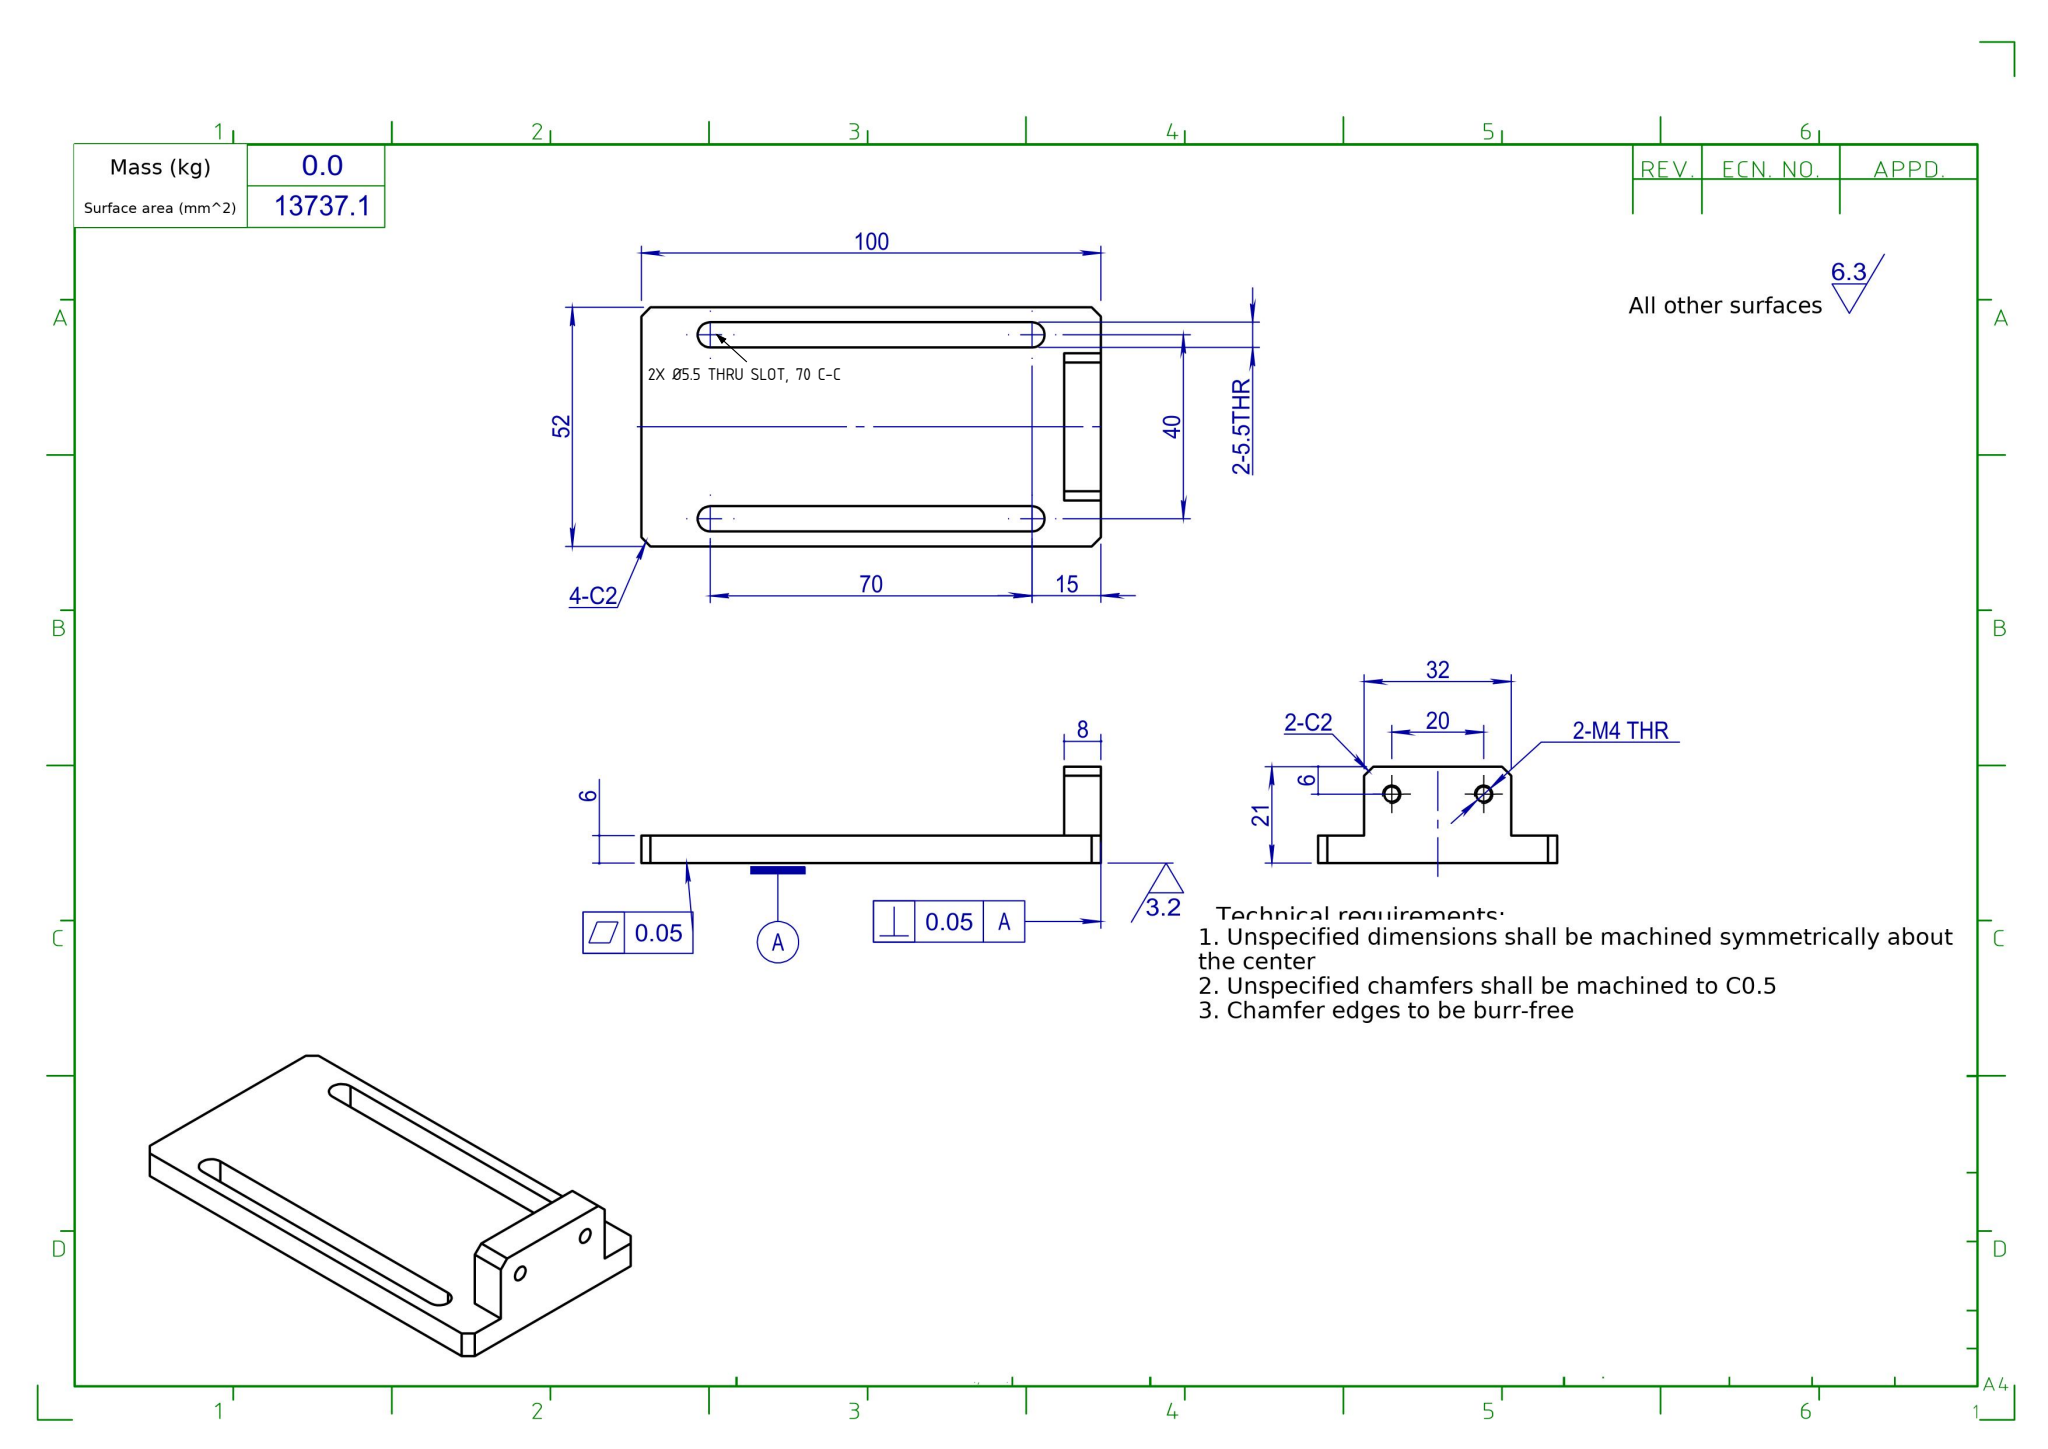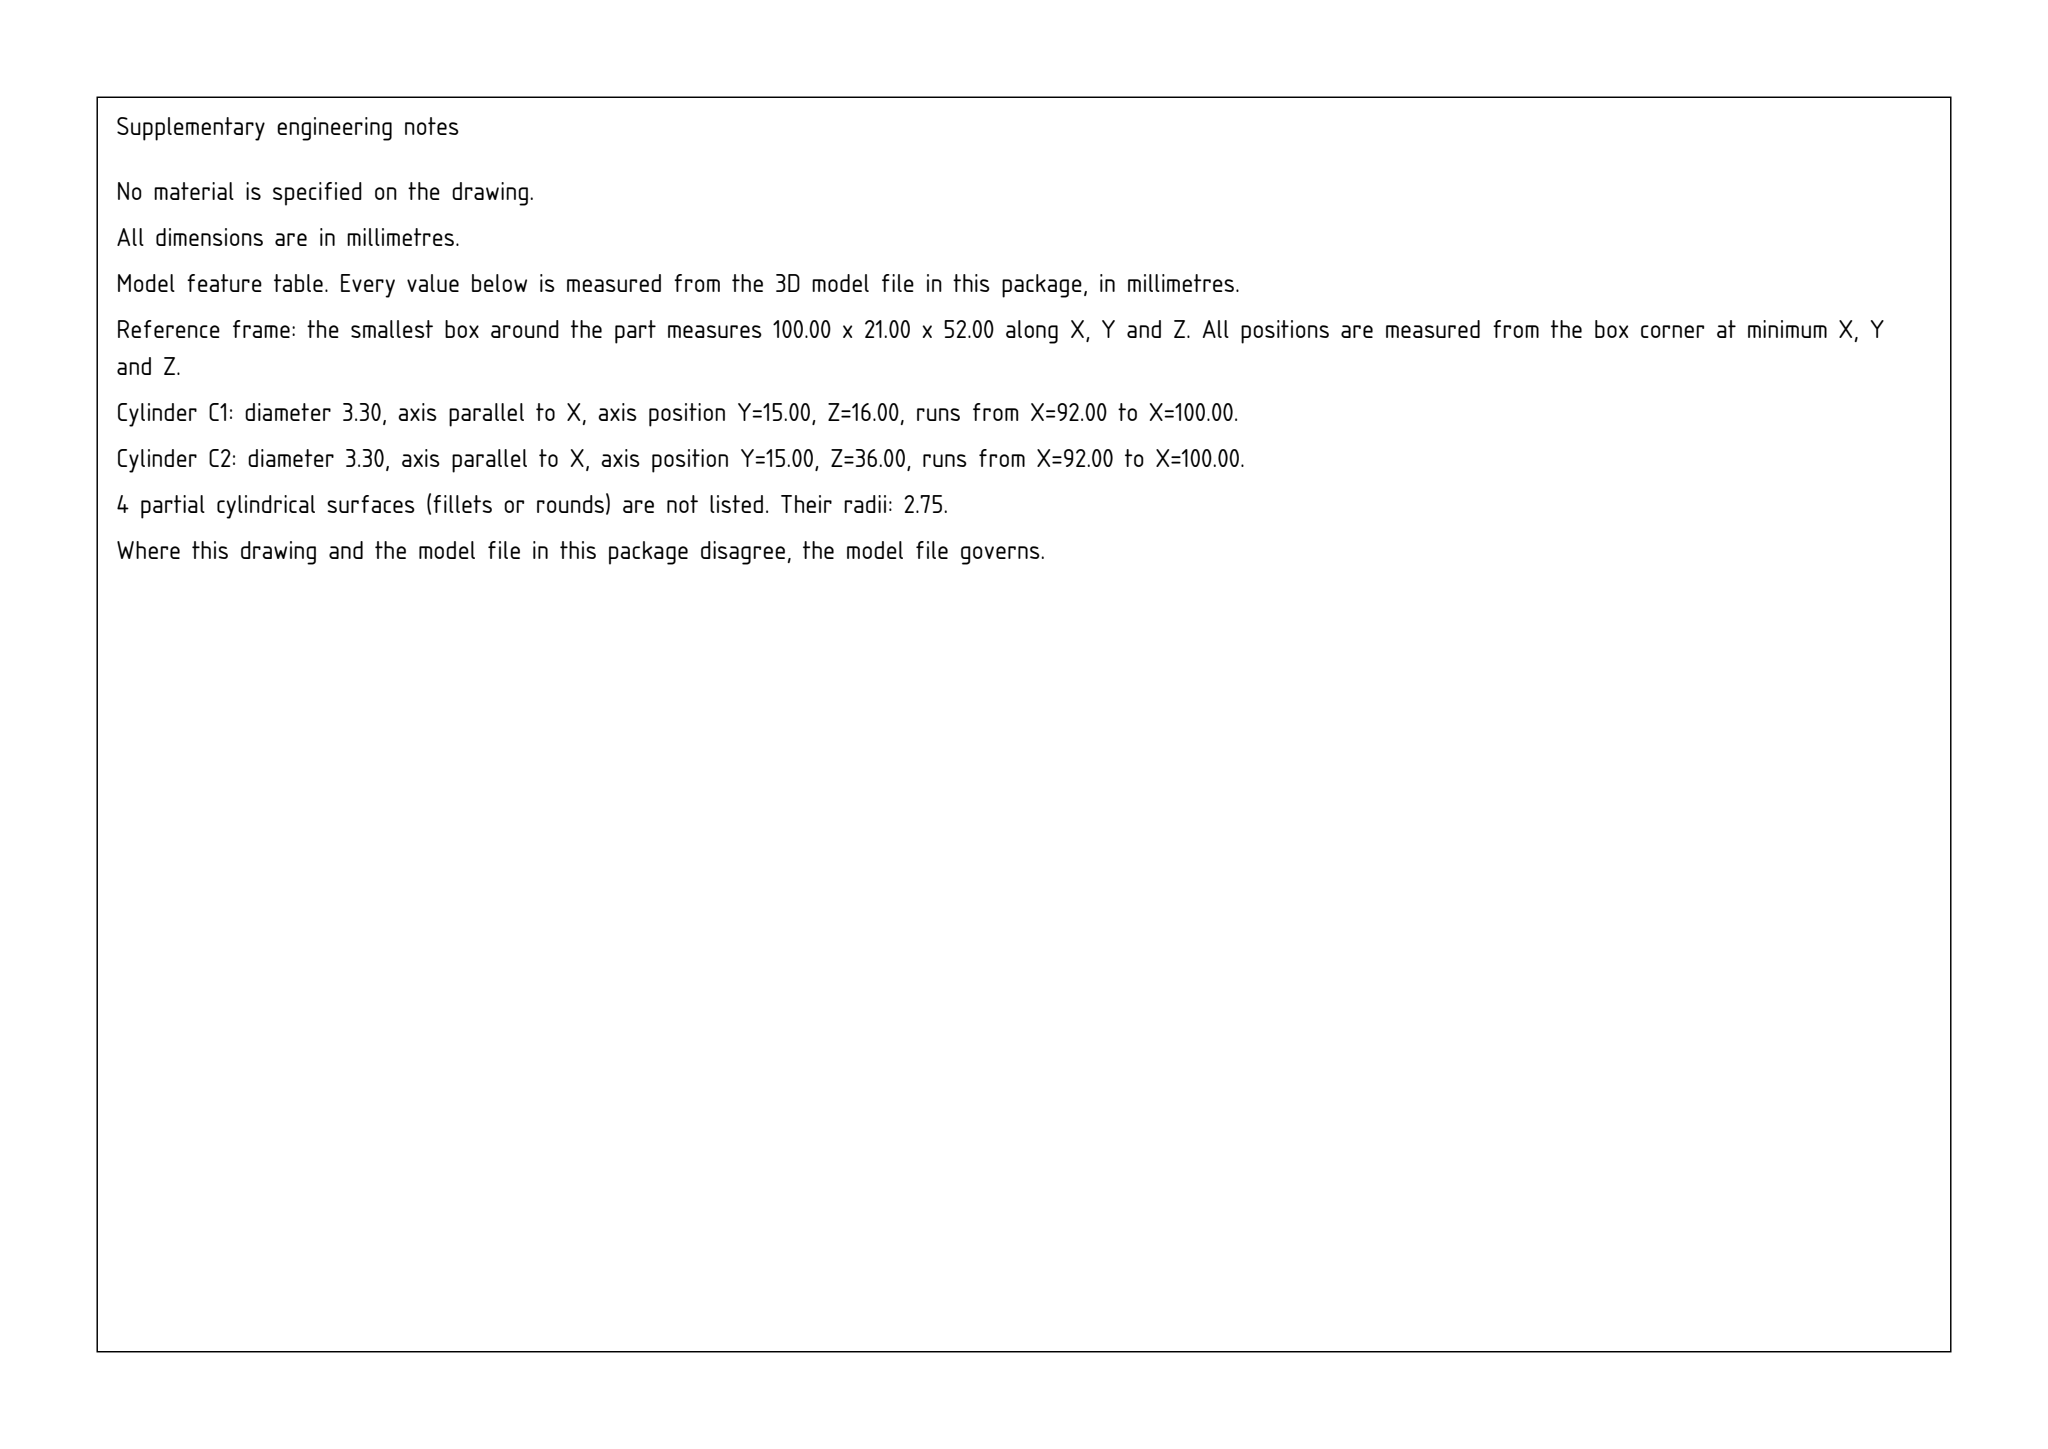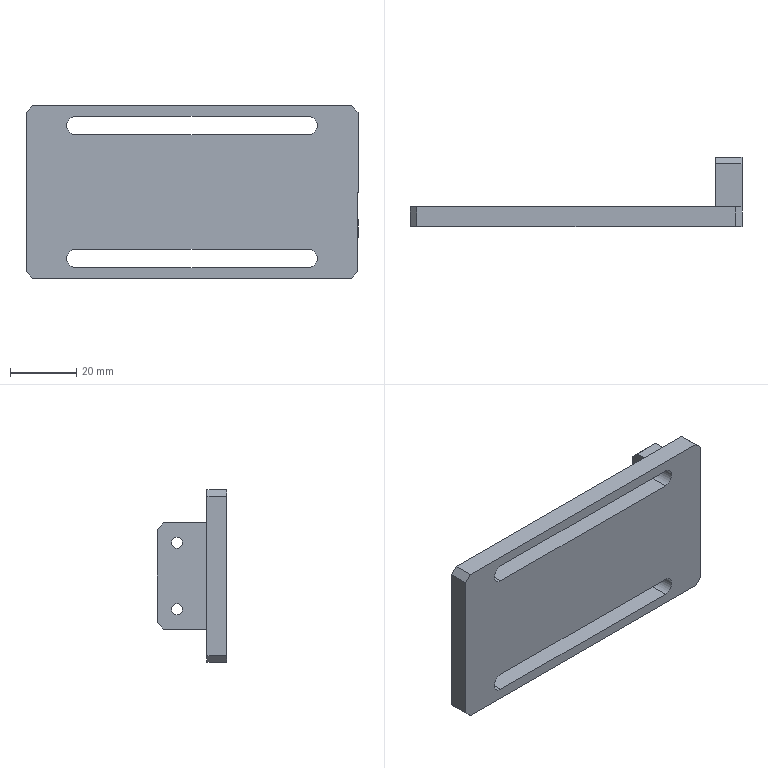Part | SolidWorks | mm | 1 solid | 28 faces | box 100 x 21 x 52 mm | volume 29918 mm3 | plane 20 | cylinder 8 | commonest cylinder face diameters 3.3 x4 5.5 x4
Drawing notes:
2-Ø5.5 THRU SLOTS, 70 LG C-C, SYM ABT CL | from the solid: Four 180° arcs Ø5.5 axis Y at x=15 & 85, z=6 & 46, from y=0 to 6 (thru 6 thk plate); slot ends 70 apart
build123d program:
from build123d import *

# Parameters (mm, degrees)
SKETCH1_W          = 100
SKETCH1_H          = 52
EXTRUDE1_DEPTH     = 3
SKETCH4_W          = 8
SKETCH4_H          = 52
EXTRUDE2_DEPTH     = 15
M4_TAPPED_HOLE1_D  = 3.3
CHAMFER1_SIZE      = 2
SKETCH9_W          = 10
SKETCH9_H          = 15
CUT_EXTRUDE3_DEPTH = 10
CHAMFER2_SIZE      = 2
CUT_EXTRUDE4_DEPTH = 59.318


with BuildPart() as part:
    # Sketch1 → Extrude1 (new, symmetric)
    with BuildSketch(Plane(origin=(0, 0, 0), x_dir=(1, 0, 0), z_dir=(0, 1, 0))):
        Rectangle(SKETCH1_W, SKETCH1_H)
    extrude(amount=EXTRUDE1_DEPTH, both=True)

    # Sketch4 → Extrude2 (add)
    with BuildSketch(Plane(origin=(0, 3, 0), x_dir=(1, 0, 0), z_dir=(0, 1, 0))):
        with Locations((46, 0)):
            Rectangle(SKETCH4_W, SKETCH4_H)
    extrude(amount=EXTRUDE2_DEPTH)

    # M4 Tapped Hole1 (through all)
    with Locations(Plane.ZY.offset(-42)):
        with Locations((-10, 12), (10, 12)):
            Hole(M4_TAPPED_HOLE1_D / 2)

    # Chamfer1
    chamfer1_edges = [part.edges().sort_by_distance(p)[0] for p in [
        (-50, 0, -26),
        (-50, 0, 26),
        (46, 18, 26),
        (46, 18, -26),
    ]]
    chamfer(chamfer1_edges, length=CHAMFER1_SIZE)

    # Sketch9 → Cut-Extrude3 (cut)
    with BuildSketch(Plane.ZY.offset(-42)):
        with Locations((-21, 10.5)):
            Rectangle(SKETCH9_W, SKETCH9_H)
        with Locations((21, 10.5)):
            Rectangle(SKETCH9_W, SKETCH9_H)
    extrude(amount=-CUT_EXTRUDE3_DEPTH, mode=Mode.SUBTRACT)

    # Chamfer2
    chamfer2_edges = [part.edges().sort_by_distance(p)[0] for p in [
        (46, 18, 16),
        (46, 18, -16),
        (50, 0, 26),
        (50, 0, -26),
    ]]
    chamfer(chamfer2_edges, length=CHAMFER2_SIZE)

    # Sketch10 → Cut-Extrude4 (cut, through all)
    with BuildSketch(Plane(origin=(0, 3, 0), x_dir=(1, 0, 0), z_dir=(0, 1, 0))):
        with BuildLine():
            Line((-35, 22.75), (35, 22.75))
            ThreePointArc((35, 22.75), (37.75, 20), (35, 17.25))
            Line((35, 17.25), (-35, 17.25))
            ThreePointArc((-35, 17.25), (-37.75, 20), (-35, 22.75))
        make_face()
        with BuildLine():
            Line((-35, -17.25), (35, -17.25))
            ThreePointArc((35, -17.25), (37.75, -20), (35, -22.75))
            Line((35, -22.75), (-35, -22.75))
            ThreePointArc((-35, -22.75), (-37.75, -20), (-35, -17.25))
        make_face()
    extrude(amount=-CUT_EXTRUDE4_DEPTH, mode=Mode.SUBTRACT)


solid = part.part
STEP:
#1=CARTESIAN_POINT('',(50.,12.,-11.65));
#2=VERTEX_POINT('',#1);
#3=CARTESIAN_POINT('',(50.,12.,-8.35));
#4=VERTEX_POINT('',#3);
#5=CARTESIAN_POINT('',(50.,12.,-10.));
#6=DIRECTION('',(-1.,0.,0.));
#7=DIRECTION('',(0.,0.,1.));
#8=AXIS2_PLACEMENT_3D('',#5,#6,#7);
#9=CIRCLE('',#8,1.65);
#10=EDGE_CURVE('',#2,#4,#9,.T.);
#11=ORIENTED_EDGE('',*,*,#10,.F.);
#12=CARTESIAN_POINT('',(42.,12.,-11.65));
#13=VERTEX_POINT('',#12);
#14=CARTESIAN_POINT('',(42.,12.,-11.65));
#15=DIRECTION('',(-1.,0.,0.));
#16=VECTOR('',#15,1000.);
#17=LINE('',#14,#16);
#18=EDGE_CURVE('',#2,#13,#17,.T.);
#19=ORIENTED_EDGE('',*,*,#18,.T.);
#20=CARTESIAN_POINT('',(42.,12.,-8.35));
#21=VERTEX_POINT('',#20);
#22=CARTESIAN_POINT('',(42.,12.,-10.));
#23=DIRECTION('',(-1.,0.,0.));
#24=DIRECTION('',(0.,0.,1.));
#25=AXIS2_PLACEMENT_3D('',#22,#23,#24);
#26=CIRCLE('',#25,1.65);
#27=EDGE_CURVE('',#13,#21,#26,.T.);
#28=ORIENTED_EDGE('',*,*,#27,.T.);
#29=CARTESIAN_POINT('',(42.,12.,-8.35));
#30=DIRECTION('',(-1.,0.,0.));
#31=VECTOR('',#30,1000.);
#32=LINE('',#29,#31);
#33=EDGE_CURVE('',#4,#21,#32,.T.);
#34=ORIENTED_EDGE('',*,*,#33,.F.);
#35=EDGE_LOOP('',(#11,#19,#28,#34));
#36=FACE_OUTER_BOUND('',#35,.T.);
#37=CARTESIAN_POINT('',(42.,12.,-10.));
#38=DIRECTION('',(-1.,0.,0.));
#39=DIRECTION('',(0.,0.,1.));
#40=AXIS2_PLACEMENT_3D('',#37,#38,#39);
#41=CYLINDRICAL_SURFACE('',#40,1.65);
#42=ADVANCED_FACE('',(#36),#41,.F.);
#43=CARTESIAN_POINT('',(50.,12.,8.35));
#44=VERTEX_POINT('',#43);
#45=CARTESIAN_POINT('',(50.,12.,11.65));
#46=VERTEX_POINT('',#45);
#47=CARTESIAN_POINT('',(50.,12.,10.));
#48=DIRECTION('',(-1.,0.,0.));
#49=DIRECTION('',(0.,0.,1.));
#50=AXIS2_PLACEMENT_3D('',#47,#48,#49);
#51=CIRCLE('',#50,1.65);
#52=EDGE_CURVE('',#44,#46,#51,.T.);
#53=ORIENTED_EDGE('',*,*,#52,.F.);
#54=CARTESIAN_POINT('',(42.,12.,8.35));
#55=VERTEX_POINT('',#54);
#56=CARTESIAN_POINT('',(42.,12.,8.35));
#57=DIRECTION('',(-1.,0.,0.));
#58=VECTOR('',#57,1000.);
#59=LINE('',#56,#58);
#60=EDGE_CURVE('',#44,#55,#59,.T.);
#61=ORIENTED_EDGE('',*,*,#60,.T.);
#62=CARTESIAN_POINT('',(42.,12.,11.65));
#63=VERTEX_POINT('',#62);
#64=CARTESIAN_POINT('',(42.,12.,10.));
#65=DIRECTION('',(-1.,0.,0.));
#66=DIRECTION('',(0.,0.,1.));
#67=AXIS2_PLACEMENT_3D('',#64,#65,#66);
#68=CIRCLE('',#67,1.65);
#69=EDGE_CURVE('',#55,#63,#68,.T.);
#70=ORIENTED_EDGE('',*,*,#69,.T.);
#71=CARTESIAN_POINT('',(42.,12.,11.65));
#72=DIRECTION('',(-1.,0.,0.));
#73=VECTOR('',#72,1000.);
#74=LINE('',#71,#73);
#75=EDGE_CURVE('',#46,#63,#74,.T.);
#76=ORIENTED_EDGE('',*,*,#75,.F.);
#77=EDGE_LOOP('',(#53,#61,#70,#76));
#78=FACE_OUTER_BOUND('',#77,.T.);
#79=CARTESIAN_POINT('',(42.,12.,10.));
#80=DIRECTION('',(-1.,0.,0.));
#81=DIRECTION('',(0.,0.,1.));
#82=AXIS2_PLACEMENT_3D('',#79,#80,#81);
#83=CYLINDRICAL_SURFACE('',#82,1.65);
#84=ADVANCED_FACE('',(#78),#83,.F.);
#85=CARTESIAN_POINT('',(-50.,3.,-24.));
#86=VERTEX_POINT('',#85);
#87=CARTESIAN_POINT('',(-50.,3.,24.));
#88=VERTEX_POINT('',#87);
#89=CARTESIAN_POINT('',(-50.,3.,-26.));
#90=DIRECTION('',(0.,0.,1.));
#91=VECTOR('',#90,1000.);
#92=LINE('',#89,#91);
#93=EDGE_CURVE('',#86,#88,#92,.T.);
#94=ORIENTED_EDGE('',*,*,#93,.F.);
#95=CARTESIAN_POINT('',(-50.,-3.,-24.));
#96=VERTEX_POINT('',#95);
#97=CARTESIAN_POINT('',(-50.,3.,-24.));
#98=DIRECTION('',(0.,-1.,0.));
#99=VECTOR('',#98,1000.);
#100=LINE('',#97,#99);
#101=EDGE_CURVE('',#86,#96,#100,.T.);
#102=ORIENTED_EDGE('',*,*,#101,.T.);
#103=CARTESIAN_POINT('',(-50.,-3.,24.));
#104=VERTEX_POINT('',#103);
#105=CARTESIAN_POINT('',(-50.,-3.,-26.));
#106=DIRECTION('',(0.,0.,1.));
#107=VECTOR('',#106,1000.);
#108=LINE('',#105,#107);
#109=EDGE_CURVE('',#96,#104,#108,.T.);
#110=ORIENTED_EDGE('',*,*,#109,.T.);
#111=CARTESIAN_POINT('',(-50.,3.,24.));
#112=DIRECTION('',(0.,1.,0.));
#113=VECTOR('',#112,1000.);
#114=LINE('',#111,#113);
#115=EDGE_CURVE('',#104,#88,#114,.T.);
#116=ORIENTED_EDGE('',*,*,#115,.T.);
#117=EDGE_LOOP('',(#94,#102,#110,#116));
#118=FACE_OUTER_BOUND('',#117,.T.);
#119=CARTESIAN_POINT('',(-50.,3.,-26.));
#120=DIRECTION('',(1.,0.,-0.));
#121=DIRECTION('',(-0.,0.,-1.));
#122=AXIS2_PLACEMENT_3D('',#119,#120,#121);
#123=PLANE('',#122);
#124=ADVANCED_FACE('',(#118),#123,.F.);
#125=CARTESIAN_POINT('',(-48.,-3.,26.));
#126=VERTEX_POINT('',#125);
#127=CARTESIAN_POINT('',(48.,-3.,26.));
#128=VERTEX_POINT('',#127);
#129=CARTESIAN_POINT('',(-50.,-3.,26.));
#130=DIRECTION('',(1.,0.,0.));
#131=VECTOR('',#130,1000.);
#132=LINE('',#129,#131);
#133=EDGE_CURVE('',#126,#128,#132,.T.);
#134=ORIENTED_EDGE('',*,*,#133,.T.);
#135=CARTESIAN_POINT('',(48.,3.,26.));
#136=VERTEX_POINT('',#135);
#137=CARTESIAN_POINT('',(48.,3.,26.));
#138=DIRECTION('',(0.,1.,0.));
#139=VECTOR('',#138,1000.);
#140=LINE('',#137,#139);
#141=EDGE_CURVE('',#128,#136,#140,.T.);
#142=ORIENTED_EDGE('',*,*,#141,.T.);
#143=CARTESIAN_POINT('',(-48.,3.,26.));
#144=VERTEX_POINT('',#143);
#145=CARTESIAN_POINT('',(-50.,3.,26.));
#146=DIRECTION('',(1.,0.,0.));
#147=VECTOR('',#146,1000.);
#148=LINE('',#145,#147);
#149=EDGE_CURVE('',#144,#136,#148,.T.);
#150=ORIENTED_EDGE('',*,*,#149,.F.);
#151=CARTESIAN_POINT('',(-48.,3.,26.));
#152=DIRECTION('',(0.,-1.,0.));
#153=VECTOR('',#152,1000.);
#154=LINE('',#151,#153);
#155=EDGE_CURVE('',#144,#126,#154,.T.);
#156=ORIENTED_EDGE('',*,*,#155,.T.);
#157=EDGE_LOOP('',(#134,#142,#150,#156));
#158=FACE_OUTER_BOUND('',#157,.T.);
#159=CARTESIAN_POINT('',(-50.,3.,26.));
#160=DIRECTION('',(0.,0.,-1.));
#161=DIRECTION('',(-1.,0.,0.));
#162=AXIS2_PLACEMENT_3D('',#159,#160,#161);
#163=PLANE('',#162);
#164=ADVANCED_FACE('',(#158),#163,.F.);
#165=CARTESIAN_POINT('',(50.,12.,-10.));
#166=DIRECTION('',(-1.,0.,0.));
#167=DIRECTION('',(0.,0.,1.));
#168=AXIS2_PLACEMENT_3D('',#165,#166,#167);
#169=CIRCLE('',#168,1.65);
#170=EDGE_CURVE('',#4,#2,#169,.T.);
#171=ORIENTED_EDGE('',*,*,#170,.T.);
#172=ORIENTED_EDGE('',*,*,#10,.T.);
#173=EDGE_LOOP('',(#171,#172));
#174=FACE_BOUND('',#173,.T.);
#175=CARTESIAN_POINT('',(50.,12.,10.));
#176=DIRECTION('',(-1.,0.,0.));
#177=DIRECTION('',(0.,0.,1.));
#178=AXIS2_PLACEMENT_3D('',#175,#176,#177);
#179=CIRCLE('',#178,1.65);
#180=EDGE_CURVE('',#46,#44,#179,.T.);
#181=ORIENTED_EDGE('',*,*,#180,.T.);
#182=ORIENTED_EDGE('',*,*,#52,.T.);
#183=EDGE_LOOP('',(#181,#182));
#184=FACE_BOUND('',#183,.T.);
#185=CARTESIAN_POINT('',(50.,18.,14.));
#186=VERTEX_POINT('',#185);
#187=CARTESIAN_POINT('',(50.,18.,-14.));
#188=VERTEX_POINT('',#187);
#189=CARTESIAN_POINT('',(50.,18.,26.));
#190=DIRECTION('',(0.,0.,-1.));
#191=VECTOR('',#190,1000.);
#192=LINE('',#189,#191);
#193=EDGE_CURVE('',#186,#188,#192,.T.);
#194=ORIENTED_EDGE('',*,*,#193,.F.);
#195=CARTESIAN_POINT('',(50.,16.,16.));
#196=VERTEX_POINT('',#195);
#197=CARTESIAN_POINT('',(50.,16.,16.));
#198=DIRECTION('',(0.,-0.7071,0.7071));
#199=VECTOR('',#198,1000.);
#200=LINE('',#197,#199);
#201=EDGE_CURVE('',#186,#196,#200,.T.);
#202=ORIENTED_EDGE('',*,*,#201,.T.);
#203=CARTESIAN_POINT('',(50.,3.,16.));
#204=VERTEX_POINT('',#203);
#205=CARTESIAN_POINT('',(50.,3.,16.));
#206=DIRECTION('',(0.,-1.,0.));
#207=VECTOR('',#206,1000.);
#208=LINE('',#205,#207);
#209=EDGE_CURVE('',#196,#204,#208,.T.);
#210=ORIENTED_EDGE('',*,*,#209,.T.);
#211=CARTESIAN_POINT('',(50.,3.,24.));
#212=VERTEX_POINT('',#211);
#213=CARTESIAN_POINT('',(50.,3.,-26.));
#214=DIRECTION('',(0.,-0.,1.));
#215=VECTOR('',#214,1000.);
#216=LINE('',#213,#215);
#217=EDGE_CURVE('',#204,#212,#216,.T.);
#218=ORIENTED_EDGE('',*,*,#217,.T.);
#219=CARTESIAN_POINT('',(50.,-3.,24.));
#220=VERTEX_POINT('',#219);
#221=CARTESIAN_POINT('',(50.,3.,24.));
#222=DIRECTION('',(0.,-1.,0.));
#223=VECTOR('',#222,1000.);
#224=LINE('',#221,#223);
#225=EDGE_CURVE('',#212,#220,#224,.T.);
#226=ORIENTED_EDGE('',*,*,#225,.T.);
#227=CARTESIAN_POINT('',(50.,-3.,-24.));
#228=VERTEX_POINT('',#227);
#229=CARTESIAN_POINT('',(50.,-3.,-26.));
#230=DIRECTION('',(-0.,0.,-1.));
#231=VECTOR('',#230,1000.);
#232=LINE('',#229,#231);
#233=EDGE_CURVE('',#220,#228,#232,.T.);
#234=ORIENTED_EDGE('',*,*,#233,.T.);
#235=CARTESIAN_POINT('',(50.,3.,-24.));
#236=VERTEX_POINT('',#235);
#237=CARTESIAN_POINT('',(50.,3.,-24.));
#238=DIRECTION('',(0.,1.,0.));
#239=VECTOR('',#238,1000.);
#240=LINE('',#237,#239);
#241=EDGE_CURVE('',#228,#236,#240,.T.);
#242=ORIENTED_EDGE('',*,*,#241,.T.);
#243=CARTESIAN_POINT('',(50.,3.,-16.));
#244=VERTEX_POINT('',#243);
#245=CARTESIAN_POINT('',(50.,3.,-26.));
#246=DIRECTION('',(0.,0.,1.));
#247=VECTOR('',#246,1000.);
#248=LINE('',#245,#247);
#249=EDGE_CURVE('',#236,#244,#248,.T.);
#250=ORIENTED_EDGE('',*,*,#249,.T.);
#251=CARTESIAN_POINT('',(50.,16.,-16.));
#252=VERTEX_POINT('',#251);
#253=CARTESIAN_POINT('',(50.,3.,-16.));
#254=DIRECTION('',(0.,1.,0.));
#255=VECTOR('',#254,1000.);
#256=LINE('',#253,#255);
#257=EDGE_CURVE('',#244,#252,#256,.T.);
#258=ORIENTED_EDGE('',*,*,#257,.T.);
#259=CARTESIAN_POINT('',(50.,18.,-14.));
#260=DIRECTION('',(0.,0.7071,0.7071));
#261=VECTOR('',#260,1000.);
#262=LINE('',#259,#261);
#263=EDGE_CURVE('',#252,#188,#262,.T.);
#264=ORIENTED_EDGE('',*,*,#263,.T.);
#265=EDGE_LOOP('',(#194,#202,#210,#218,#226,#234,#242,#250,#258,#264));
#266=FACE_OUTER_BOUND('',#265,.T.);
#267=CARTESIAN_POINT('',(50.,3.,-26.));
#268=DIRECTION('',(-1.,0.,0.));
#269=DIRECTION('',(0.,0.,1.));
#270=AXIS2_PLACEMENT_3D('',#267,#268,#269);
#271=PLANE('',#270);
#272=ADVANCED_FACE('',(#174,#184,#266),#271,.F.);
#273=CARTESIAN_POINT('',(48.,3.,-26.));
#274=VERTEX_POINT('',#273);
#275=CARTESIAN_POINT('',(-48.,3.,-26.));
#276=VERTEX_POINT('',#275);
#277=CARTESIAN_POINT('',(-50.,3.,-26.));
#278=DIRECTION('',(-1.,0.,0.));
#279=VECTOR('',#278,1000.);
#280=LINE('',#277,#279);
#281=EDGE_CURVE('',#274,#276,#280,.T.);
#282=ORIENTED_EDGE('',*,*,#281,.F.);
#283=CARTESIAN_POINT('',(48.,-3.,-26.));
#284=VERTEX_POINT('',#283);
#285=CARTESIAN_POINT('',(48.,3.,-26.));
#286=DIRECTION('',(0.,-1.,0.));
#287=VECTOR('',#286,1000.);
#288=LINE('',#285,#287);
#289=EDGE_CURVE('',#274,#284,#288,.T.);
#290=ORIENTED_EDGE('',*,*,#289,.T.);
#291=CARTESIAN_POINT('',(-48.,-3.,-26.));
#292=VERTEX_POINT('',#291);
#293=CARTESIAN_POINT('',(-50.,-3.,-26.));
#294=DIRECTION('',(-1.,0.,0.));
#295=VECTOR('',#294,1000.);
#296=LINE('',#293,#295);
#297=EDGE_CURVE('',#284,#292,#296,.T.);
#298=ORIENTED_EDGE('',*,*,#297,.T.);
#299=CARTESIAN_POINT('',(-48.,3.,-26.));
#300=DIRECTION('',(0.,1.,0.));
#301=VECTOR('',#300,1000.);
#302=LINE('',#299,#301);
#303=EDGE_CURVE('',#292,#276,#302,.T.);
#304=ORIENTED_EDGE('',*,*,#303,.T.);
#305=EDGE_LOOP('',(#282,#290,#298,#304));
#306=FACE_OUTER_BOUND('',#305,.T.);
#307=CARTESIAN_POINT('',(-50.,3.,-26.));
#308=DIRECTION('',(0.,0.,1.));
#309=DIRECTION('',(1.,0.,0.));
#310=AXIS2_PLACEMENT_3D('',#307,#308,#309);
#311=PLANE('',#310);
#312=ADVANCED_FACE('',(#306),#311,.F.);
#313=CARTESIAN_POINT('',(35.,3.,22.75));
#314=VERTEX_POINT('',#313);
#315=CARTESIAN_POINT('',(35.,3.,17.25));
#316=VERTEX_POINT('',#315);
#317=CARTESIAN_POINT('',(35.,3.,20.));
#318=DIRECTION('',(0.,1.,0.));
#319=DIRECTION('',(0.,0.,-1.));
#320=AXIS2_PLACEMENT_3D('',#317,#318,#319);
#321=CIRCLE('',#320,2.75);
#322=EDGE_CURVE('',#314,#316,#321,.T.);
#323=ORIENTED_EDGE('',*,*,#322,.F.);
#324=CARTESIAN_POINT('',(-35.,3.,22.75));
#325=VERTEX_POINT('',#324);
#326=CARTESIAN_POINT('',(-35.,3.,22.75));
#327=DIRECTION('',(1.,0.,0.));
#328=VECTOR('',#327,1000.);
#329=LINE('',#326,#328);
#330=EDGE_CURVE('',#325,#314,#329,.T.);
#331=ORIENTED_EDGE('',*,*,#330,.F.);
#332=CARTESIAN_POINT('',(-35.,3.,17.25));
#333=VERTEX_POINT('',#332);
#334=CARTESIAN_POINT('',(-35.,3.,20.));
#335=DIRECTION('',(0.,1.,0.));
#336=DIRECTION('',(0.,0.,-1.));
#337=AXIS2_PLACEMENT_3D('',#334,#335,#336);
#338=CIRCLE('',#337,2.75);
#339=EDGE_CURVE('',#333,#325,#338,.T.);
#340=ORIENTED_EDGE('',*,*,#339,.F.);
#341=CARTESIAN_POINT('',(-35.,3.,17.25));
#342=DIRECTION('',(-1.,0.,0.));
#343=VECTOR('',#342,1000.);
#344=LINE('',#341,#343);
#345=EDGE_CURVE('',#316,#333,#344,.T.);
#346=ORIENTED_EDGE('',*,*,#345,.F.);
#347=EDGE_LOOP('',(#323,#331,#340,#346));
#348=FACE_BOUND('',#347,.T.);
#349=CARTESIAN_POINT('',(-35.,3.,-22.75));
#350=VERTEX_POINT('',#349);
#351=CARTESIAN_POINT('',(-35.,3.,-17.25));
#352=VERTEX_POINT('',#351);
#353=CARTESIAN_POINT('',(-35.,3.,-20.));
#354=DIRECTION('',(0.,1.,0.));
#355=DIRECTION('',(0.,0.,1.));
#356=AXIS2_PLACEMENT_3D('',#353,#354,#355);
#357=CIRCLE('',#356,2.75);
#358=EDGE_CURVE('',#350,#352,#357,.T.);
#359=ORIENTED_EDGE('',*,*,#358,.F.);
#360=CARTESIAN_POINT('',(35.,3.,-22.75));
#361=VERTEX_POINT('',#360);
#362=CARTESIAN_POINT('',(-35.,3.,-22.75));
#363=DIRECTION('',(-1.,0.,0.));
#364=VECTOR('',#363,1000.);
#365=LINE('',#362,#364);
#366=EDGE_CURVE('',#361,#350,#365,.T.);
#367=ORIENTED_EDGE('',*,*,#366,.F.);
#368=CARTESIAN_POINT('',(35.,3.,-17.25));
#369=VERTEX_POINT('',#368);
#370=CARTESIAN_POINT('',(35.,3.,-20.));
#371=DIRECTION('',(0.,1.,0.));
#372=DIRECTION('',(0.,0.,1.));
#373=AXIS2_PLACEMENT_3D('',#370,#371,#372);
#374=CIRCLE('',#373,2.75);
#375=EDGE_CURVE('',#369,#361,#374,.T.);
#376=ORIENTED_EDGE('',*,*,#375,.F.);
#377=CARTESIAN_POINT('',(-35.,3.,-17.25));
#378=DIRECTION('',(1.,0.,0.));
#379=VECTOR('',#378,1000.);
#380=LINE('',#377,#379);
#381=EDGE_CURVE('',#352,#369,#380,.T.);
#382=ORIENTED_EDGE('',*,*,#381,.F.);
#383=EDGE_LOOP('',(#359,#367,#376,#382));
#384=FACE_BOUND('',#383,.T.);
#385=ORIENTED_EDGE('',*,*,#149,.T.);
#386=CARTESIAN_POINT('',(-1.,3.,75.));
#387=DIRECTION('',(0.7071,0.,-0.7071));
#388=VECTOR('',#387,1000.);
#389=LINE('',#386,#388);
#390=EDGE_CURVE('',#136,#212,#389,.T.);
#391=ORIENTED_EDGE('',*,*,#390,.T.);
#392=ORIENTED_EDGE('',*,*,#217,.F.);
#393=CARTESIAN_POINT('',(42.,3.,16.));
#394=VERTEX_POINT('',#393);
#395=CARTESIAN_POINT('',(52.,3.,16.));
#396=DIRECTION('',(-1.,0.,0.));
#397=VECTOR('',#396,1000.);
#398=LINE('',#395,#397);
#399=EDGE_CURVE('',#204,#394,#398,.T.);
#400=ORIENTED_EDGE('',*,*,#399,.T.);
#401=CARTESIAN_POINT('',(42.,3.,-16.));
#402=VERTEX_POINT('',#401);
#403=CARTESIAN_POINT('',(42.,3.,26.));
#404=DIRECTION('',(0.,0.,1.));
#405=VECTOR('',#404,1000.);
#406=LINE('',#403,#405);
#407=EDGE_CURVE('',#402,#394,#406,.T.);
#408=ORIENTED_EDGE('',*,*,#407,.F.);
#409=CARTESIAN_POINT('',(52.,3.,-16.));
#410=DIRECTION('',(-1.,0.,0.));
#411=VECTOR('',#410,1000.);
#412=LINE('',#409,#411);
#413=EDGE_CURVE('',#244,#402,#412,.T.);
#414=ORIENTED_EDGE('',*,*,#413,.F.);
#415=ORIENTED_EDGE('',*,*,#249,.F.);
#416=CARTESIAN_POINT('',(25.,3.,-49.));
#417=DIRECTION('',(-0.7071,0.,-0.7071));
#418=VECTOR('',#417,1000.);
#419=LINE('',#416,#418);
#420=EDGE_CURVE('',#236,#274,#419,.T.);
#421=ORIENTED_EDGE('',*,*,#420,.T.);
#422=ORIENTED_EDGE('',*,*,#281,.T.);
#423=CARTESIAN_POINT('',(-75.,3.,1.));
#424=DIRECTION('',(-0.7071,0.,0.7071));
#425=VECTOR('',#424,1000.);
#426=LINE('',#423,#425);
#427=EDGE_CURVE('',#276,#86,#426,.T.);
#428=ORIENTED_EDGE('',*,*,#427,.T.);
#429=ORIENTED_EDGE('',*,*,#93,.T.);
#430=CARTESIAN_POINT('',(-49.,3.,25.));
#431=DIRECTION('',(0.7071,0.,0.7071));
#432=VECTOR('',#431,1000.);
#433=LINE('',#430,#432);
#434=EDGE_CURVE('',#88,#144,#433,.T.);
#435=ORIENTED_EDGE('',*,*,#434,.T.);
#436=EDGE_LOOP('',(#385,#391,#392,#400,#408,#414,#415,#421,#422,#428,#429,#435));
#437=FACE_OUTER_BOUND('',#436,.T.);
#438=CARTESIAN_POINT('',(-50.,3.,26.));
#439=DIRECTION('',(0.,1.,0.));
#440=DIRECTION('',(0.,0.,1.));
#441=AXIS2_PLACEMENT_3D('',#438,#439,#440);
#442=PLANE('',#441);
#443=ADVANCED_FACE('',(#348,#384,#437),#442,.T.);
#444=CARTESIAN_POINT('',(-35.,-3.,22.75));
#445=VERTEX_POINT('',#444);
#446=CARTESIAN_POINT('',(35.,-3.,22.75));
#447=VERTEX_POINT('',#446);
#448=CARTESIAN_POINT('',(-35.,-3.,22.75));
#449=DIRECTION('',(1.,0.,0.));
#450=VECTOR('',#449,1000.);
#451=LINE('',#448,#450);
#452=EDGE_CURVE('',#445,#447,#451,.T.);
#453=ORIENTED_EDGE('',*,*,#452,.T.);
#454=CARTESIAN_POINT('',(35.,-3.,17.25));
#455=VERTEX_POINT('',#454);
#456=CARTESIAN_POINT('',(35.,-3.,20.));
#457=DIRECTION('',(0.,1.,0.));
#458=DIRECTION('',(0.,0.,-1.));
#459=AXIS2_PLACEMENT_3D('',#456,#457,#458);
#460=CIRCLE('',#459,2.75);
#461=EDGE_CURVE('',#447,#455,#460,.T.);
#462=ORIENTED_EDGE('',*,*,#461,.T.);
#463=CARTESIAN_POINT('',(-35.,-3.,17.25));
#464=VERTEX_POINT('',#463);
#465=CARTESIAN_POINT('',(-35.,-3.,17.25));
#466=DIRECTION('',(-1.,0.,0.));
#467=VECTOR('',#466,1000.);
#468=LINE('',#465,#467);
#469=EDGE_CURVE('',#455,#464,#468,.T.);
#470=ORIENTED_EDGE('',*,*,#469,.T.);
#471=CARTESIAN_POINT('',(-35.,-3.,20.));
#472=DIRECTION('',(0.,1.,0.));
#473=DIRECTION('',(0.,0.,-1.));
#474=AXIS2_PLACEMENT_3D('',#471,#472,#473);
#475=CIRCLE('',#474,2.75);
#476=EDGE_CURVE('',#464,#445,#475,.T.);
#477=ORIENTED_EDGE('',*,*,#476,.T.);
#478=EDGE_LOOP('',(#453,#462,#470,#477));
#479=FACE_BOUND('',#478,.T.);
#480=CARTESIAN_POINT('',(35.,-3.,-22.75));
#481=VERTEX_POINT('',#480);
#482=CARTESIAN_POINT('',(-35.,-3.,-22.75));
#483=VERTEX_POINT('',#482);
#484=CARTESIAN_POINT('',(-35.,-3.,-22.75));
#485=DIRECTION('',(-1.,0.,0.));
#486=VECTOR('',#485,1000.);
#487=LINE('',#484,#486);
#488=EDGE_CURVE('',#481,#483,#487,.T.);
#489=ORIENTED_EDGE('',*,*,#488,.T.);
#490=CARTESIAN_POINT('',(-35.,-3.,-17.25));
#491=VERTEX_POINT('',#490);
#492=CARTESIAN_POINT('',(-35.,-3.,-20.));
#493=DIRECTION('',(0.,1.,0.));
#494=DIRECTION('',(0.,0.,1.));
#495=AXIS2_PLACEMENT_3D('',#492,#493,#494);
#496=CIRCLE('',#495,2.75);
#497=EDGE_CURVE('',#483,#491,#496,.T.);
#498=ORIENTED_EDGE('',*,*,#497,.T.);
#499=CARTESIAN_POINT('',(35.,-3.,-17.25));
#500=VERTEX_POINT('',#499);
#501=CARTESIAN_POINT('',(-35.,-3.,-17.25));
#502=DIRECTION('',(1.,0.,0.));
#503=VECTOR('',#502,1000.);
#504=LINE('',#501,#503);
#505=EDGE_CURVE('',#491,#500,#504,.T.);
#506=ORIENTED_EDGE('',*,*,#505,.T.);
#507=CARTESIAN_POINT('',(35.,-3.,-20.));
#508=DIRECTION('',(0.,1.,0.));
#509=DIRECTION('',(0.,0.,1.));
#510=AXIS2_PLACEMENT_3D('',#507,#508,#509);
#511=CIRCLE('',#510,2.75);
#512=EDGE_CURVE('',#500,#481,#511,.T.);
#513=ORIENTED_EDGE('',*,*,#512,.T.);
#514=EDGE_LOOP('',(#489,#498,#506,#513));
#515=FACE_BOUND('',#514,.T.);
#516=ORIENTED_EDGE('',*,*,#233,.F.);
#517=CARTESIAN_POINT('',(50.,-3.,24.));
#518=DIRECTION('',(-0.7071,0.,0.7071));
#519=VECTOR('',#518,1000.);
#520=LINE('',#517,#519);
#521=EDGE_CURVE('',#220,#128,#520,.T.);
#522=ORIENTED_EDGE('',*,*,#521,.T.);
#523=ORIENTED_EDGE('',*,*,#133,.F.);
#524=CARTESIAN_POINT('',(-48.,-3.,26.));
#525=DIRECTION('',(-0.7071,0.,-0.7071));
#526=VECTOR('',#525,1000.);
#527=LINE('',#524,#526);
#528=EDGE_CURVE('',#126,#104,#527,.T.);
#529=ORIENTED_EDGE('',*,*,#528,.T.);
#530=ORIENTED_EDGE('',*,*,#109,.F.);
#531=CARTESIAN_POINT('',(-50.,-3.,-24.));
#532=DIRECTION('',(0.7071,0.,-0.7071));
#533=VECTOR('',#532,1000.);
#534=LINE('',#531,#533);
#535=EDGE_CURVE('',#96,#292,#534,.T.);
#536=ORIENTED_EDGE('',*,*,#535,.T.);
#537=ORIENTED_EDGE('',*,*,#297,.F.);
#538=CARTESIAN_POINT('',(48.,-3.,-26.));
#539=DIRECTION('',(0.7071,0.,0.7071));
#540=VECTOR('',#539,1000.);
#541=LINE('',#538,#540);
#542=EDGE_CURVE('',#284,#228,#541,.T.);
#543=ORIENTED_EDGE('',*,*,#542,.T.);
#544=EDGE_LOOP('',(#516,#522,#523,#529,#530,#536,#537,#543));
#545=FACE_OUTER_BOUND('',#544,.T.);
#546=CARTESIAN_POINT('',(-50.,-3.,26.));
#547=DIRECTION('',(0.,1.,0.));
#548=DIRECTION('',(0.,0.,1.));
#549=AXIS2_PLACEMENT_3D('',#546,#547,#548);
#550=PLANE('',#549);
#551=ADVANCED_FACE('',(#479,#515,#545),#550,.F.);
#552=CARTESIAN_POINT('',(42.,12.,-10.));
#553=DIRECTION('',(-1.,0.,0.));
#554=DIRECTION('',(0.,0.,1.));
#555=AXIS2_PLACEMENT_3D('',#552,#553,#554);
#556=CIRCLE('',#555,1.65);
#557=EDGE_CURVE('',#21,#13,#556,.T.);
#558=ORIENTED_EDGE('',*,*,#557,.F.);
#559=ORIENTED_EDGE('',*,*,#27,.F.);
#560=EDGE_LOOP('',(#558,#559));
#561=FACE_BOUND('',#560,.T.);
#562=CARTESIAN_POINT('',(42.,12.,10.));
#563=DIRECTION('',(-1.,0.,0.));
#564=DIRECTION('',(0.,0.,1.));
#565=AXIS2_PLACEMENT_3D('',#562,#563,#564);
#566=CIRCLE('',#565,1.65);
#567=EDGE_CURVE('',#63,#55,#566,.T.);
#568=ORIENTED_EDGE('',*,*,#567,.F.);
#569=ORIENTED_EDGE('',*,*,#69,.F.);
#570=EDGE_LOOP('',(#568,#569));
#571=FACE_BOUND('',#570,.T.);
#572=CARTESIAN_POINT('',(42.,16.,16.));
#573=VERTEX_POINT('',#572);
#574=CARTESIAN_POINT('',(42.,3.,16.));
#575=DIRECTION('',(0.,-1.,0.));
#576=VECTOR('',#575,1000.);
#577=LINE('',#574,#576);
#578=EDGE_CURVE('',#573,#394,#577,.T.);
#579=ORIENTED_EDGE('',*,*,#578,.F.);
#580=CARTESIAN_POINT('',(42.,18.,14.));
#581=VERTEX_POINT('',#580);
#582=CARTESIAN_POINT('',(42.,16.,16.));
#583=DIRECTION('',(-0.,0.7071,-0.7071));
#584=VECTOR('',#583,1000.);
#585=LINE('',#582,#584);
#586=EDGE_CURVE('',#573,#581,#585,.T.);
#587=ORIENTED_EDGE('',*,*,#586,.T.);
#588=CARTESIAN_POINT('',(42.,18.,-14.));
#589=VERTEX_POINT('',#588);
#590=CARTESIAN_POINT('',(42.,18.,26.));
#591=DIRECTION('',(0.,0.,1.));
#592=VECTOR('',#591,1000.);
#593=LINE('',#590,#592);
#594=EDGE_CURVE('',#589,#581,#593,.T.);
#595=ORIENTED_EDGE('',*,*,#594,.F.);
#596=CARTESIAN_POINT('',(42.,16.,-16.));
#597=VERTEX_POINT('',#596);
#598=CARTESIAN_POINT('',(42.,18.,-14.));
#599=DIRECTION('',(-0.,-0.7071,-0.7071));
#600=VECTOR('',#599,1000.);
#601=LINE('',#598,#600);
#602=EDGE_CURVE('',#589,#597,#601,.T.);
#603=ORIENTED_EDGE('',*,*,#602,.T.);
#604=CARTESIAN_POINT('',(42.,3.,-16.));
#605=DIRECTION('',(0.,1.,0.));
#606=VECTOR('',#605,1000.);
#607=LINE('',#604,#606);
#608=EDGE_CURVE('',#402,#597,#607,.T.);
#609=ORIENTED_EDGE('',*,*,#608,.F.);
#610=ORIENTED_EDGE('',*,*,#407,.T.);
#611=EDGE_LOOP('',(#579,#587,#595,#603,#609,#610));
#612=FACE_OUTER_BOUND('',#611,.T.);
#613=CARTESIAN_POINT('',(42.,18.,26.));
#614=DIRECTION('',(1.,0.,-0.));
#615=DIRECTION('',(-0.,0.,-1.));
#616=AXIS2_PLACEMENT_3D('',#613,#614,#615);
#617=PLANE('',#616);
#618=ADVANCED_FACE('',(#561,#571,#612),#617,.F.);
#619=ORIENTED_EDGE('',*,*,#594,.T.);
#620=CARTESIAN_POINT('',(50.,18.,14.));
#621=DIRECTION('',(1.,0.,0.));
#622=VECTOR('',#621,1000.);
#623=LINE('',#620,#622);
#624=EDGE_CURVE('',#581,#186,#623,.T.);
#625=ORIENTED_EDGE('',*,*,#624,.T.);
#626=ORIENTED_EDGE('',*,*,#193,.T.);
#627=CARTESIAN_POINT('',(42.,18.,-14.));
#628=DIRECTION('',(-1.,0.,0.));
#629=VECTOR('',#628,1000.);
#630=LINE('',#627,#629);
#631=EDGE_CURVE('',#188,#589,#630,.T.);
#632=ORIENTED_EDGE('',*,*,#631,.T.);
#633=EDGE_LOOP('',(#619,#625,#626,#632));
#634=FACE_OUTER_BOUND('',#633,.T.);
#635=CARTESIAN_POINT('',(50.,18.,-26.));
#636=DIRECTION('',(0.,1.,0.));
#637=DIRECTION('',(0.,0.,1.));
#638=AXIS2_PLACEMENT_3D('',#635,#636,#637);
#639=PLANE('',#638);
#640=ADVANCED_FACE('',(#634),#639,.T.);
#641=ORIENTED_EDGE('',*,*,#60,.F.);
#642=ORIENTED_EDGE('',*,*,#180,.F.);
#643=ORIENTED_EDGE('',*,*,#75,.T.);
#644=ORIENTED_EDGE('',*,*,#567,.T.);
#645=EDGE_LOOP('',(#641,#642,#643,#644));
#646=FACE_OUTER_BOUND('',#645,.T.);
#647=CARTESIAN_POINT('',(42.,12.,10.));
#648=DIRECTION('',(-1.,0.,0.));
#649=DIRECTION('',(0.,0.,1.));
#650=AXIS2_PLACEMENT_3D('',#647,#648,#649);
#651=CYLINDRICAL_SURFACE('',#650,1.65);
#652=ADVANCED_FACE('',(#646),#651,.F.);
#653=ORIENTED_EDGE('',*,*,#18,.F.);
#654=ORIENTED_EDGE('',*,*,#170,.F.);
#655=ORIENTED_EDGE('',*,*,#33,.T.);
#656=ORIENTED_EDGE('',*,*,#557,.T.);
#657=EDGE_LOOP('',(#653,#654,#655,#656));
#658=FACE_OUTER_BOUND('',#657,.T.);
#659=CARTESIAN_POINT('',(42.,12.,-10.));
#660=DIRECTION('',(-1.,0.,0.));
#661=DIRECTION('',(0.,0.,1.));
#662=AXIS2_PLACEMENT_3D('',#659,#660,#661);
#663=CYLINDRICAL_SURFACE('',#662,1.65);
#664=ADVANCED_FACE('',(#658),#663,.F.);
#665=ORIENTED_EDGE('',*,*,#427,.F.);
#666=ORIENTED_EDGE('',*,*,#303,.F.);
#667=ORIENTED_EDGE('',*,*,#535,.F.);
#668=ORIENTED_EDGE('',*,*,#101,.F.);
#669=EDGE_LOOP('',(#665,#666,#667,#668));
#670=FACE_OUTER_BOUND('',#669,.T.);
#671=CARTESIAN_POINT('',(-50.,3.,-24.));
#672=DIRECTION('',(0.7071,0.,0.7071));
#673=DIRECTION('',(0.7071,0.,-0.7071));
#674=AXIS2_PLACEMENT_3D('',#671,#672,#673);
#675=PLANE('',#674);
#676=ADVANCED_FACE('',(#670),#675,.F.);
#677=ORIENTED_EDGE('',*,*,#434,.F.);
#678=ORIENTED_EDGE('',*,*,#115,.F.);
#679=ORIENTED_EDGE('',*,*,#528,.F.);
#680=ORIENTED_EDGE('',*,*,#155,.F.);
#681=EDGE_LOOP('',(#677,#678,#679,#680));
#682=FACE_OUTER_BOUND('',#681,.T.);
#683=CARTESIAN_POINT('',(-48.,3.,26.));
#684=DIRECTION('',(0.7071,0.,-0.7071));
#685=DIRECTION('',(-0.7071,0.,-0.7071));
#686=AXIS2_PLACEMENT_3D('',#683,#684,#685);
#687=PLANE('',#686);
#688=ADVANCED_FACE('',(#682),#687,.F.);
#689=ORIENTED_EDGE('',*,*,#608,.T.);
#690=CARTESIAN_POINT('',(50.,16.,-16.));
#691=DIRECTION('',(1.,0.,0.));
#692=VECTOR('',#691,1000.);
#693=LINE('',#690,#692);
#694=EDGE_CURVE('',#597,#252,#693,.T.);
#695=ORIENTED_EDGE('',*,*,#694,.T.);
#696=ORIENTED_EDGE('',*,*,#257,.F.);
#697=ORIENTED_EDGE('',*,*,#413,.T.);
#698=EDGE_LOOP('',(#689,#695,#696,#697));
#699=FACE_OUTER_BOUND('',#698,.T.);
#700=CARTESIAN_POINT('',(52.,3.,-16.));
#701=DIRECTION('',(0.,0.,1.));
#702=DIRECTION('',(1.,0.,0.));
#703=AXIS2_PLACEMENT_3D('',#700,#701,#702);
#704=PLANE('',#703);
#705=ADVANCED_FACE('',(#699),#704,.F.);
#706=ORIENTED_EDGE('',*,*,#209,.F.);
#707=CARTESIAN_POINT('',(42.,16.,16.));
#708=DIRECTION('',(-1.,0.,0.));
#709=VECTOR('',#708,1000.);
#710=LINE('',#707,#709);
#711=EDGE_CURVE('',#196,#573,#710,.T.);
#712=ORIENTED_EDGE('',*,*,#711,.T.);
#713=ORIENTED_EDGE('',*,*,#578,.T.);
#714=ORIENTED_EDGE('',*,*,#399,.F.);
#715=EDGE_LOOP('',(#706,#712,#713,#714));
#716=FACE_OUTER_BOUND('',#715,.T.);
#717=CARTESIAN_POINT('',(52.,3.,16.));
#718=DIRECTION('',(0.,0.,-1.));
#719=DIRECTION('',(-1.,0.,0.));
#720=AXIS2_PLACEMENT_3D('',#717,#718,#719);
#721=PLANE('',#720);
#722=ADVANCED_FACE('',(#716),#721,.F.);
#723=ORIENTED_EDGE('',*,*,#201,.F.);
#724=ORIENTED_EDGE('',*,*,#624,.F.);
#725=ORIENTED_EDGE('',*,*,#586,.F.);
#726=ORIENTED_EDGE('',*,*,#711,.F.);
#727=EDGE_LOOP('',(#723,#724,#725,#726));
#728=FACE_OUTER_BOUND('',#727,.T.);
#729=CARTESIAN_POINT('',(52.,16.,16.));
#730=DIRECTION('',(0.,0.7071,0.7071));
#731=DIRECTION('',(1.,0.,0.));
#732=AXIS2_PLACEMENT_3D('',#729,#730,#731);
#733=PLANE('',#732);
#734=ADVANCED_FACE('',(#728),#733,.T.);
#735=ORIENTED_EDGE('',*,*,#263,.F.);
#736=ORIENTED_EDGE('',*,*,#694,.F.);
#737=ORIENTED_EDGE('',*,*,#602,.F.);
#738=ORIENTED_EDGE('',*,*,#631,.F.);
#739=EDGE_LOOP('',(#735,#736,#737,#738));
#740=FACE_OUTER_BOUND('',#739,.T.);
#741=CARTESIAN_POINT('',(50.,18.,-14.));
#742=DIRECTION('',(0.,0.7071,-0.7071));
#743=DIRECTION('',(1.,0.,0.));
#744=AXIS2_PLACEMENT_3D('',#741,#742,#743);
#745=PLANE('',#744);
#746=ADVANCED_FACE('',(#740),#745,.T.);
#747=ORIENTED_EDGE('',*,*,#390,.F.);
#748=ORIENTED_EDGE('',*,*,#141,.F.);
#749=ORIENTED_EDGE('',*,*,#521,.F.);
#750=ORIENTED_EDGE('',*,*,#225,.F.);
#751=EDGE_LOOP('',(#747,#748,#749,#750));
#752=FACE_OUTER_BOUND('',#751,.T.);
#753=CARTESIAN_POINT('',(50.,3.,24.));
#754=DIRECTION('',(-0.7071,0.,-0.7071));
#755=DIRECTION('',(0.,-1.,0.));
#756=AXIS2_PLACEMENT_3D('',#753,#754,#755);
#757=PLANE('',#756);
#758=ADVANCED_FACE('',(#752),#757,.F.);
#759=ORIENTED_EDGE('',*,*,#420,.F.);
#760=ORIENTED_EDGE('',*,*,#241,.F.);
#761=ORIENTED_EDGE('',*,*,#542,.F.);
#762=ORIENTED_EDGE('',*,*,#289,.F.);
#763=EDGE_LOOP('',(#759,#760,#761,#762));
#764=FACE_OUTER_BOUND('',#763,.T.);
#765=CARTESIAN_POINT('',(48.,3.,-26.));
#766=DIRECTION('',(-0.7071,0.,0.7071));
#767=DIRECTION('',(0.,-1.,0.));
#768=AXIS2_PLACEMENT_3D('',#765,#766,#767);
#769=PLANE('',#768);
#770=ADVANCED_FACE('',(#764),#769,.F.);
#771=ORIENTED_EDGE('',*,*,#358,.T.);
#772=CARTESIAN_POINT('',(-35.,-3.,-17.25));
#773=DIRECTION('',(0.,1.,0.));
#774=VECTOR('',#773,1000.);
#775=LINE('',#772,#774);
#776=EDGE_CURVE('',#491,#352,#775,.T.);
#777=ORIENTED_EDGE('',*,*,#776,.F.);
#778=ORIENTED_EDGE('',*,*,#497,.F.);
#779=CARTESIAN_POINT('',(-35.,-3.,-22.75));
#780=DIRECTION('',(0.,1.,0.));
#781=VECTOR('',#780,1000.);
#782=LINE('',#779,#781);
#783=EDGE_CURVE('',#483,#350,#782,.T.);
#784=ORIENTED_EDGE('',*,*,#783,.T.);
#785=EDGE_LOOP('',(#771,#777,#778,#784));
#786=FACE_OUTER_BOUND('',#785,.T.);
#787=CARTESIAN_POINT('',(-35.,-3.,-20.));
#788=DIRECTION('',(0.,1.,0.));
#789=DIRECTION('',(0.,0.,1.));
#790=AXIS2_PLACEMENT_3D('',#787,#788,#789);
#791=CYLINDRICAL_SURFACE('',#790,2.75);
#792=ADVANCED_FACE('',(#786),#791,.F.);
#793=ORIENTED_EDGE('',*,*,#366,.T.);
#794=ORIENTED_EDGE('',*,*,#783,.F.);
#795=ORIENTED_EDGE('',*,*,#488,.F.);
#796=CARTESIAN_POINT('',(35.,-3.,-22.75));
#797=DIRECTION('',(0.,1.,0.));
#798=VECTOR('',#797,1000.);
#799=LINE('',#796,#798);
#800=EDGE_CURVE('',#481,#361,#799,.T.);
#801=ORIENTED_EDGE('',*,*,#800,.T.);
#802=EDGE_LOOP('',(#793,#794,#795,#801));
#803=FACE_OUTER_BOUND('',#802,.T.);
#804=CARTESIAN_POINT('',(-35.,-3.,-22.75));
#805=DIRECTION('',(0.,0.,-1.));
#806=DIRECTION('',(-1.,0.,0.));
#807=AXIS2_PLACEMENT_3D('',#804,#805,#806);
#808=PLANE('',#807);
#809=ADVANCED_FACE('',(#803),#808,.F.);
#810=ORIENTED_EDGE('',*,*,#375,.T.);
#811=ORIENTED_EDGE('',*,*,#800,.F.);
#812=ORIENTED_EDGE('',*,*,#512,.F.);
#813=CARTESIAN_POINT('',(35.,-3.,-17.25));
#814=DIRECTION('',(0.,1.,0.));
#815=VECTOR('',#814,1000.);
#816=LINE('',#813,#815);
#817=EDGE_CURVE('',#500,#369,#816,.T.);
#818=ORIENTED_EDGE('',*,*,#817,.T.);
#819=EDGE_LOOP('',(#810,#811,#812,#818));
#820=FACE_OUTER_BOUND('',#819,.T.);
#821=CARTESIAN_POINT('',(35.,-3.,-20.));
#822=DIRECTION('',(0.,1.,0.));
#823=DIRECTION('',(0.,0.,1.));
#824=AXIS2_PLACEMENT_3D('',#821,#822,#823);
#825=CYLINDRICAL_SURFACE('',#824,2.75);
#826=ADVANCED_FACE('',(#820),#825,.F.);
#827=ORIENTED_EDGE('',*,*,#381,.T.);
#828=ORIENTED_EDGE('',*,*,#817,.F.);
#829=ORIENTED_EDGE('',*,*,#505,.F.);
#830=ORIENTED_EDGE('',*,*,#776,.T.);
#831=EDGE_LOOP('',(#827,#828,#829,#830));
#832=FACE_OUTER_BOUND('',#831,.T.);
#833=CARTESIAN_POINT('',(-35.,-3.,-17.25));
#834=DIRECTION('',(0.,0.,1.));
#835=DIRECTION('',(1.,0.,0.));
#836=AXIS2_PLACEMENT_3D('',#833,#834,#835);
#837=PLANE('',#836);
#838=ADVANCED_FACE('',(#832),#837,.F.);
#839=ORIENTED_EDGE('',*,*,#322,.T.);
#840=CARTESIAN_POINT('',(35.,-3.,17.25));
#841=DIRECTION('',(0.,1.,0.));
#842=VECTOR('',#841,1000.);
#843=LINE('',#840,#842);
#844=EDGE_CURVE('',#455,#316,#843,.T.);
#845=ORIENTED_EDGE('',*,*,#844,.F.);
#846=ORIENTED_EDGE('',*,*,#461,.F.);
#847=CARTESIAN_POINT('',(35.,-3.,22.75));
#848=DIRECTION('',(0.,1.,0.));
#849=VECTOR('',#848,1000.);
#850=LINE('',#847,#849);
#851=EDGE_CURVE('',#447,#314,#850,.T.);
#852=ORIENTED_EDGE('',*,*,#851,.T.);
#853=EDGE_LOOP('',(#839,#845,#846,#852));
#854=FACE_OUTER_BOUND('',#853,.T.);
#855=CARTESIAN_POINT('',(35.,-3.,20.));
#856=DIRECTION('',(0.,1.,0.));
#857=DIRECTION('',(0.,0.,1.));
#858=AXIS2_PLACEMENT_3D('',#855,#856,#857);
#859=CYLINDRICAL_SURFACE('',#858,2.75);
#860=ADVANCED_FACE('',(#854),#859,.F.);
#861=ORIENTED_EDGE('',*,*,#330,.T.);
#862=ORIENTED_EDGE('',*,*,#851,.F.);
#863=ORIENTED_EDGE('',*,*,#452,.F.);
#864=CARTESIAN_POINT('',(-35.,-3.,22.75));
#865=DIRECTION('',(0.,1.,0.));
#866=VECTOR('',#865,1000.);
#867=LINE('',#864,#866);
#868=EDGE_CURVE('',#445,#325,#867,.T.);
#869=ORIENTED_EDGE('',*,*,#868,.T.);
#870=EDGE_LOOP('',(#861,#862,#863,#869));
#871=FACE_OUTER_BOUND('',#870,.T.);
#872=CARTESIAN_POINT('',(-35.,-3.,22.75));
#873=DIRECTION('',(0.,0.,1.));
#874=DIRECTION('',(1.,0.,0.));
#875=AXIS2_PLACEMENT_3D('',#872,#873,#874);
#876=PLANE('',#875);
#877=ADVANCED_FACE('',(#871),#876,.F.);
#878=ORIENTED_EDGE('',*,*,#339,.T.);
#879=ORIENTED_EDGE('',*,*,#868,.F.);
#880=ORIENTED_EDGE('',*,*,#476,.F.);
#881=CARTESIAN_POINT('',(-35.,-3.,17.25));
#882=DIRECTION('',(0.,1.,0.));
#883=VECTOR('',#882,1000.);
#884=LINE('',#881,#883);
#885=EDGE_CURVE('',#464,#333,#884,.T.);
#886=ORIENTED_EDGE('',*,*,#885,.T.);
#887=EDGE_LOOP('',(#878,#879,#880,#886));
#888=FACE_OUTER_BOUND('',#887,.T.);
#889=CARTESIAN_POINT('',(-35.,-3.,20.));
#890=DIRECTION('',(0.,1.,0.));
#891=DIRECTION('',(0.,0.,1.));
#892=AXIS2_PLACEMENT_3D('',#889,#890,#891);
#893=CYLINDRICAL_SURFACE('',#892,2.75);
#894=ADVANCED_FACE('',(#888),#893,.F.);
#895=ORIENTED_EDGE('',*,*,#345,.T.);
#896=ORIENTED_EDGE('',*,*,#885,.F.);
#897=ORIENTED_EDGE('',*,*,#469,.F.);
#898=ORIENTED_EDGE('',*,*,#844,.T.);
#899=EDGE_LOOP('',(#895,#896,#897,#898));
#900=FACE_OUTER_BOUND('',#899,.T.);
#901=CARTESIAN_POINT('',(-35.,-3.,17.25));
#902=DIRECTION('',(0.,0.,-1.));
#903=DIRECTION('',(-1.,0.,0.));
#904=AXIS2_PLACEMENT_3D('',#901,#902,#903);
#905=PLANE('',#904);
#906=ADVANCED_FACE('',(#900),#905,.F.);
#907=CLOSED_SHELL('',(#42,#84,#124,#164,#272,#312,#443,#551,#618,#640,#652,#664,#676,#688,#705,#722,#734,#746,#758,#770,#792,#809,#826,#838,#860,#877,#894,#906));
#908=MANIFOLD_SOLID_BREP('',#907);
#909=CARTESIAN_POINT('',(0.,0.,0.));
#910=DIRECTION('',(0.,0.,1.));
#911=DIRECTION('',(1.,0.,0.));
#912=AXIS2_PLACEMENT_3D('',#909,#910,#911);
#913=(LENGTH_UNIT()NAMED_UNIT(*)SI_UNIT(.MILLI.,.METRE.));
#914=UNCERTAINTY_MEASURE_WITH_UNIT(LENGTH_MEASURE(0.00001),#913,'','');
#915=(NAMED_UNIT(*)PLANE_ANGLE_UNIT()SI_UNIT($,.RADIAN.));
#916=(NAMED_UNIT(*)SI_UNIT($,.STERADIAN.)SOLID_ANGLE_UNIT());
#917=(GEOMETRIC_REPRESENTATION_CONTEXT(3)GLOBAL_UNCERTAINTY_ASSIGNED_CONTEXT((#914))GLOBAL_UNIT_ASSIGNED_CONTEXT((#913,#915,#916))REPRESENTATION_CONTEXT('',''));
#918=ADVANCED_BREP_SHAPE_REPRESENTATION('',(#908,#912),#917);